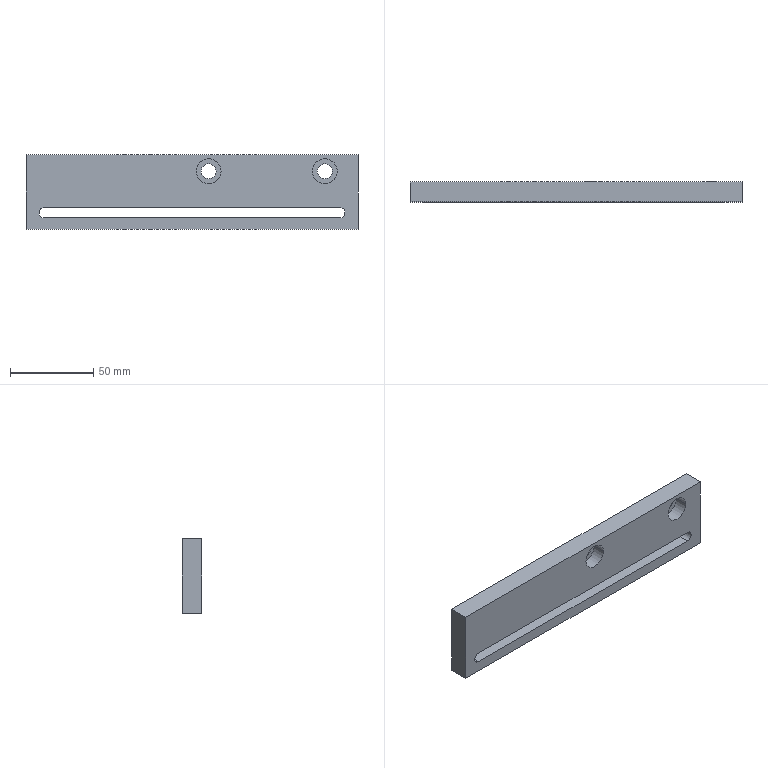Component | SolidWorks | SL021-102-4096.SL4PRT-1 | 1 solid | 21 faces | box 200 x 12 x 45 mm | volume 90833 mm3 | cylinder 11 | plane 10 | commonest cylinder face diameters 15 x4 9 x4 6.3 x3 | material AL6061
build123d program:
from build123d import *

# Parameters (mm, degrees)
SKETCH1_W                                          = 200
SKETCH1_H                                          = 45
BOSS_EXTRUDE1_DEPTH                                = 6
HOLE_SIZE_ACCORDING_TO_TYPE_1_OF_HEXAG_D           = 9
HOLE_SIZE_ACCORDING_TO_TYPE_1_OF_HEXAG_CBORE_D     = 15
HOLE_SIZE_ACCORDING_TO_TYPE_1_OF_HEXAG_CBORE_DEPTH = 8
CUT_EXTRUDE1_DEPTH                                 = 104.2


with BuildPart() as part:
    # Sketch1 → Boss-Extrude1 (new, symmetric)
    with BuildSketch(Plane.XY):
        Rectangle(SKETCH1_W, SKETCH1_H)
    extrude(amount=BOSS_EXTRUDE1_DEPTH, both=True)

    # Hole Size _According to_ Type 1 of Hexag (through all)
    with Locations(Plane(origin=(0, 0, 6), x_dir=(-1, 0, 0), z_dir=(0, 0, 1))):
        with Locations((-10, -12.5), (-80, -12.5)):
            CounterBoreHole(HOLE_SIZE_ACCORDING_TO_TYPE_1_OF_HEXAG_D / 2, HOLE_SIZE_ACCORDING_TO_TYPE_1_OF_HEXAG_CBORE_D / 2, HOLE_SIZE_ACCORDING_TO_TYPE_1_OF_HEXAG_CBORE_DEPTH)

    # Sketch4 → Cut-Extrude1 (cut, through all)
    with BuildSketch(Plane(origin=(0, 0, -6), x_dir=(-1, 0, 0), z_dir=(0, 0, -1))):
        with BuildLine():
            Line((-89, -9.35), (89, -9.35))
            ThreePointArc((89, -9.35), (92.15, -12.5), (89, -15.65))
            Line((89, -15.65), (-89, -15.65))
            ThreePointArc((-89, -15.65), (-92.15, -12.5), (-89, -9.35))
        make_face()
    extrude(amount=-CUT_EXTRUDE1_DEPTH, mode=Mode.SUBTRACT)


solid = part.part

# Placed as in the assembly
solid = solid.moved(Location((-136.163, -96.499, -318.878), (90, 0, 0)))
STEP:
#1=COLOUR_RGB('',0.7922,0.8196,0.9333);
#2=FILL_AREA_STYLE_COLOUR('',#1);
#3=FILL_AREA_STYLE('',(#2));
#4=SURFACE_STYLE_FILL_AREA(#3);
#5=SURFACE_SIDE_STYLE('',(#4));
#6=SURFACE_STYLE_USAGE(.BOTH.,#5);
#7=PRESENTATION_STYLE_ASSIGNMENT((#6));
#8=CARTESIAN_POINT('',(-8.989,-4.035,-13.046));
#9=VERTEX_POINT('',#8);
#10=CARTESIAN_POINT('',(-8.865,-4.035,-12.922));
#11=VERTEX_POINT('',#10);
#12=CARTESIAN_POINT('',(-8.865,-4.035,-13.046));
#13=DIRECTION('',(-0.,1.,-0.));
#14=DIRECTION('',(-1.,0.,0.));
#15=AXIS2_PLACEMENT_3D('',#12,#13,#14);
#16=CIRCLE('',#15,0.124);
#17=EDGE_CURVE('',#9,#11,#16,.T.);
#18=ORIENTED_EDGE('',*,*,#17,.F.);
#19=CARTESIAN_POINT('',(-8.989,-3.563,-13.046));
#20=VERTEX_POINT('',#19);
#21=CARTESIAN_POINT('',(-8.989,-4.035,-13.046));
#22=DIRECTION('',(-0.,1.,-0.));
#23=VECTOR('',#22,39.37);
#24=LINE('',#21,#23);
#25=EDGE_CURVE('',#9,#20,#24,.T.);
#26=ORIENTED_EDGE('',*,*,#25,.T.);
#27=CARTESIAN_POINT('',(-8.865,-3.563,-12.922));
#28=VERTEX_POINT('',#27);
#29=CARTESIAN_POINT('',(-8.865,-3.563,-13.046));
#30=DIRECTION('',(-0.,1.,-0.));
#31=DIRECTION('',(-1.,0.,0.));
#32=AXIS2_PLACEMENT_3D('',#29,#30,#31);
#33=CIRCLE('',#32,0.124);
#34=EDGE_CURVE('',#20,#28,#33,.T.);
#35=ORIENTED_EDGE('',*,*,#34,.T.);
#36=CARTESIAN_POINT('',(-8.865,-4.035,-12.922));
#37=DIRECTION('',(-0.,1.,-0.));
#38=VECTOR('',#37,39.37);
#39=LINE('',#36,#38);
#40=EDGE_CURVE('',#11,#28,#39,.T.);
#41=ORIENTED_EDGE('',*,*,#40,.F.);
#42=EDGE_LOOP('',(#18,#26,#35,#41));
#43=FACE_OUTER_BOUND('',#42,.T.);
#44=CARTESIAN_POINT('',(-8.865,-4.035,-13.046));
#45=DIRECTION('',(-0.,1.,-0.));
#46=DIRECTION('',(-1.,0.,0.));
#47=AXIS2_PLACEMENT_3D('',#44,#45,#46);
#48=CYLINDRICAL_SURFACE('',#47,0.124);
#49=ADVANCED_FACE('',(#43),#48,.F.);
#50=CARTESIAN_POINT('',(-5.262,-3.72,-12.062));
#51=VERTEX_POINT('',#50);
#52=CARTESIAN_POINT('',(-4.672,-3.72,-12.062));
#53=VERTEX_POINT('',#52);
#54=CARTESIAN_POINT('',(-4.967,-3.72,-12.062));
#55=DIRECTION('',(0.,-1.,0.));
#56=DIRECTION('',(1.,0.,0.));
#57=AXIS2_PLACEMENT_3D('',#54,#55,#56);
#58=CIRCLE('',#57,0.2953);
#59=EDGE_CURVE('',#51,#53,#58,.T.);
#60=ORIENTED_EDGE('',*,*,#59,.F.);
#61=CARTESIAN_POINT('',(-5.262,-4.035,-12.062));
#62=VERTEX_POINT('',#61);
#63=CARTESIAN_POINT('',(-5.262,-4.035,-12.062));
#64=DIRECTION('',(0.,-1.,0.));
#65=VECTOR('',#64,39.37);
#66=LINE('',#63,#65);
#67=EDGE_CURVE('',#51,#62,#66,.T.);
#68=ORIENTED_EDGE('',*,*,#67,.T.);
#69=CARTESIAN_POINT('',(-4.672,-4.035,-12.062));
#70=VERTEX_POINT('',#69);
#71=CARTESIAN_POINT('',(-4.967,-4.035,-12.062));
#72=DIRECTION('',(0.,-1.,0.));
#73=DIRECTION('',(1.,0.,0.));
#74=AXIS2_PLACEMENT_3D('',#71,#72,#73);
#75=CIRCLE('',#74,0.2953);
#76=EDGE_CURVE('',#62,#70,#75,.T.);
#77=ORIENTED_EDGE('',*,*,#76,.T.);
#78=CARTESIAN_POINT('',(-4.672,-4.035,-12.062));
#79=DIRECTION('',(0.,-1.,0.));
#80=VECTOR('',#79,39.37);
#81=LINE('',#78,#80);
#82=EDGE_CURVE('',#53,#70,#81,.T.);
#83=ORIENTED_EDGE('',*,*,#82,.F.);
#84=EDGE_LOOP('',(#60,#68,#77,#83));
#85=FACE_OUTER_BOUND('',#84,.T.);
#86=CARTESIAN_POINT('',(-4.967,-4.035,-12.062));
#87=DIRECTION('',(0.,-1.,0.));
#88=DIRECTION('',(1.,0.,0.));
#89=AXIS2_PLACEMENT_3D('',#86,#87,#88);
#90=CYLINDRICAL_SURFACE('',#89,0.2953);
#91=ADVANCED_FACE('',(#85),#90,.F.);
#92=CARTESIAN_POINT('',(-5.144,-3.563,-12.062));
#93=VERTEX_POINT('',#92);
#94=CARTESIAN_POINT('',(-4.79,-3.563,-12.062));
#95=VERTEX_POINT('',#94);
#96=CARTESIAN_POINT('',(-4.967,-3.563,-12.062));
#97=DIRECTION('',(0.,-1.,0.));
#98=DIRECTION('',(1.,0.,0.));
#99=AXIS2_PLACEMENT_3D('',#96,#97,#98);
#100=CIRCLE('',#99,0.1772);
#101=EDGE_CURVE('',#93,#95,#100,.T.);
#102=ORIENTED_EDGE('',*,*,#101,.F.);
#103=CARTESIAN_POINT('',(-5.144,-3.72,-12.062));
#104=VERTEX_POINT('',#103);
#105=CARTESIAN_POINT('',(-5.144,-4.035,-12.062));
#106=DIRECTION('',(0.,-1.,0.));
#107=VECTOR('',#106,39.37);
#108=LINE('',#105,#107);
#109=EDGE_CURVE('',#93,#104,#108,.T.);
#110=ORIENTED_EDGE('',*,*,#109,.T.);
#111=CARTESIAN_POINT('',(-4.79,-3.72,-12.062));
#112=VERTEX_POINT('',#111);
#113=CARTESIAN_POINT('',(-4.967,-3.72,-12.062));
#114=DIRECTION('',(0.,-1.,0.));
#115=DIRECTION('',(1.,0.,0.));
#116=AXIS2_PLACEMENT_3D('',#113,#114,#115);
#117=CIRCLE('',#116,0.1772);
#118=EDGE_CURVE('',#104,#112,#117,.T.);
#119=ORIENTED_EDGE('',*,*,#118,.T.);
#120=CARTESIAN_POINT('',(-4.79,-4.035,-12.062));
#121=DIRECTION('',(0.,-1.,0.));
#122=VECTOR('',#121,39.37);
#123=LINE('',#120,#122);
#124=EDGE_CURVE('',#95,#112,#123,.T.);
#125=ORIENTED_EDGE('',*,*,#124,.F.);
#126=EDGE_LOOP('',(#102,#110,#119,#125));
#127=FACE_OUTER_BOUND('',#126,.T.);
#128=CARTESIAN_POINT('',(-4.967,-4.035,-12.062));
#129=DIRECTION('',(0.,-1.,0.));
#130=DIRECTION('',(1.,0.,0.));
#131=AXIS2_PLACEMENT_3D('',#128,#129,#130);
#132=CYLINDRICAL_SURFACE('',#131,0.1772);
#133=ADVANCED_FACE('',(#127),#132,.F.);
#134=CARTESIAN_POINT('',(-2.506,-3.72,-12.062));
#135=VERTEX_POINT('',#134);
#136=CARTESIAN_POINT('',(-1.916,-3.72,-12.062));
#137=VERTEX_POINT('',#136);
#138=CARTESIAN_POINT('',(-2.211,-3.72,-12.062));
#139=DIRECTION('',(0.,-1.,0.));
#140=DIRECTION('',(1.,0.,0.));
#141=AXIS2_PLACEMENT_3D('',#138,#139,#140);
#142=CIRCLE('',#141,0.2953);
#143=EDGE_CURVE('',#135,#137,#142,.T.);
#144=ORIENTED_EDGE('',*,*,#143,.F.);
#145=CARTESIAN_POINT('',(-2.506,-4.035,-12.062));
#146=VERTEX_POINT('',#145);
#147=CARTESIAN_POINT('',(-2.506,-4.035,-12.062));
#148=DIRECTION('',(0.,-1.,0.));
#149=VECTOR('',#148,39.37);
#150=LINE('',#147,#149);
#151=EDGE_CURVE('',#135,#146,#150,.T.);
#152=ORIENTED_EDGE('',*,*,#151,.T.);
#153=CARTESIAN_POINT('',(-1.916,-4.035,-12.062));
#154=VERTEX_POINT('',#153);
#155=CARTESIAN_POINT('',(-2.211,-4.035,-12.062));
#156=DIRECTION('',(0.,-1.,0.));
#157=DIRECTION('',(1.,0.,0.));
#158=AXIS2_PLACEMENT_3D('',#155,#156,#157);
#159=CIRCLE('',#158,0.2953);
#160=EDGE_CURVE('',#146,#154,#159,.T.);
#161=ORIENTED_EDGE('',*,*,#160,.T.);
#162=CARTESIAN_POINT('',(-1.916,-4.035,-12.062));
#163=DIRECTION('',(0.,-1.,0.));
#164=VECTOR('',#163,39.37);
#165=LINE('',#162,#164);
#166=EDGE_CURVE('',#137,#154,#165,.T.);
#167=ORIENTED_EDGE('',*,*,#166,.F.);
#168=EDGE_LOOP('',(#144,#152,#161,#167));
#169=FACE_OUTER_BOUND('',#168,.T.);
#170=CARTESIAN_POINT('',(-2.211,-4.035,-12.062));
#171=DIRECTION('',(0.,-1.,0.));
#172=DIRECTION('',(1.,0.,0.));
#173=AXIS2_PLACEMENT_3D('',#170,#171,#172);
#174=CYLINDRICAL_SURFACE('',#173,0.2953);
#175=ADVANCED_FACE('',(#169),#174,.F.);
#176=CARTESIAN_POINT('',(-2.388,-3.563,-12.062));
#177=VERTEX_POINT('',#176);
#178=CARTESIAN_POINT('',(-2.034,-3.563,-12.062));
#179=VERTEX_POINT('',#178);
#180=CARTESIAN_POINT('',(-2.211,-3.563,-12.062));
#181=DIRECTION('',(0.,-1.,0.));
#182=DIRECTION('',(1.,0.,0.));
#183=AXIS2_PLACEMENT_3D('',#180,#181,#182);
#184=CIRCLE('',#183,0.1772);
#185=EDGE_CURVE('',#177,#179,#184,.T.);
#186=ORIENTED_EDGE('',*,*,#185,.F.);
#187=CARTESIAN_POINT('',(-2.388,-3.72,-12.062));
#188=VERTEX_POINT('',#187);
#189=CARTESIAN_POINT('',(-2.388,-4.035,-12.062));
#190=DIRECTION('',(0.,-1.,0.));
#191=VECTOR('',#190,39.37);
#192=LINE('',#189,#191);
#193=EDGE_CURVE('',#177,#188,#192,.T.);
#194=ORIENTED_EDGE('',*,*,#193,.T.);
#195=CARTESIAN_POINT('',(-2.034,-3.72,-12.062));
#196=VERTEX_POINT('',#195);
#197=CARTESIAN_POINT('',(-2.211,-3.72,-12.062));
#198=DIRECTION('',(0.,-1.,0.));
#199=DIRECTION('',(1.,0.,0.));
#200=AXIS2_PLACEMENT_3D('',#197,#198,#199);
#201=CIRCLE('',#200,0.1772);
#202=EDGE_CURVE('',#188,#196,#201,.T.);
#203=ORIENTED_EDGE('',*,*,#202,.T.);
#204=CARTESIAN_POINT('',(-2.034,-4.035,-12.062));
#205=DIRECTION('',(0.,-1.,0.));
#206=VECTOR('',#205,39.37);
#207=LINE('',#204,#206);
#208=EDGE_CURVE('',#179,#196,#207,.T.);
#209=ORIENTED_EDGE('',*,*,#208,.F.);
#210=EDGE_LOOP('',(#186,#194,#203,#209));
#211=FACE_OUTER_BOUND('',#210,.T.);
#212=CARTESIAN_POINT('',(-2.211,-4.035,-12.062));
#213=DIRECTION('',(0.,-1.,0.));
#214=DIRECTION('',(1.,0.,0.));
#215=AXIS2_PLACEMENT_3D('',#212,#213,#214);
#216=CYLINDRICAL_SURFACE('',#215,0.1772);
#217=ADVANCED_FACE('',(#211),#216,.F.);
#218=CARTESIAN_POINT('',(-1.424,-3.563,-13.44));
#219=VERTEX_POINT('',#218);
#220=CARTESIAN_POINT('',(-1.424,-3.563,-11.668));
#221=VERTEX_POINT('',#220);
#222=CARTESIAN_POINT('',(-1.424,-3.563,-13.44));
#223=DIRECTION('',(-0.,0.,1.));
#224=VECTOR('',#223,39.37);
#225=LINE('',#222,#224);
#226=EDGE_CURVE('',#219,#221,#225,.T.);
#227=ORIENTED_EDGE('',*,*,#226,.T.);
#228=CARTESIAN_POINT('',(-1.424,-4.035,-11.668));
#229=VERTEX_POINT('',#228);
#230=CARTESIAN_POINT('',(-1.424,-4.035,-11.668));
#231=DIRECTION('',(-0.,1.,-0.));
#232=VECTOR('',#231,39.37);
#233=LINE('',#230,#232);
#234=EDGE_CURVE('',#229,#221,#233,.T.);
#235=ORIENTED_EDGE('',*,*,#234,.F.);
#236=CARTESIAN_POINT('',(-1.424,-4.035,-13.44));
#237=VERTEX_POINT('',#236);
#238=CARTESIAN_POINT('',(-1.424,-4.035,-13.44));
#239=DIRECTION('',(-0.,0.,1.));
#240=VECTOR('',#239,39.37);
#241=LINE('',#238,#240);
#242=EDGE_CURVE('',#237,#229,#241,.T.);
#243=ORIENTED_EDGE('',*,*,#242,.F.);
#244=CARTESIAN_POINT('',(-1.424,-4.035,-13.44));
#245=DIRECTION('',(-0.,1.,-0.));
#246=VECTOR('',#245,39.37);
#247=LINE('',#244,#246);
#248=EDGE_CURVE('',#237,#219,#247,.T.);
#249=ORIENTED_EDGE('',*,*,#248,.T.);
#250=EDGE_LOOP('',(#227,#235,#243,#249));
#251=FACE_OUTER_BOUND('',#250,.T.);
#252=CARTESIAN_POINT('',(-1.424,-4.035,-13.44));
#253=DIRECTION('',(-1.,-0.,-0.));
#254=DIRECTION('',(0.,-1.,0.));
#255=AXIS2_PLACEMENT_3D('',#252,#253,#254);
#256=PLANE('',#255);
#257=ADVANCED_FACE('',(#251),#256,.F.);
#258=CARTESIAN_POINT('',(-9.298,-3.563,-11.668));
#259=VERTEX_POINT('',#258);
#260=CARTESIAN_POINT('',(-9.298,-3.563,-11.668));
#261=DIRECTION('',(-1.,-0.,-0.));
#262=VECTOR('',#261,39.37);
#263=LINE('',#260,#262);
#264=EDGE_CURVE('',#221,#259,#263,.T.);
#265=ORIENTED_EDGE('',*,*,#264,.T.);
#266=CARTESIAN_POINT('',(-9.298,-4.035,-11.668));
#267=VERTEX_POINT('',#266);
#268=CARTESIAN_POINT('',(-9.298,-4.035,-11.668));
#269=DIRECTION('',(-0.,1.,-0.));
#270=VECTOR('',#269,39.37);
#271=LINE('',#268,#270);
#272=EDGE_CURVE('',#267,#259,#271,.T.);
#273=ORIENTED_EDGE('',*,*,#272,.F.);
#274=CARTESIAN_POINT('',(-9.298,-4.035,-11.668));
#275=DIRECTION('',(-1.,-0.,-0.));
#276=VECTOR('',#275,39.37);
#277=LINE('',#274,#276);
#278=EDGE_CURVE('',#229,#267,#277,.T.);
#279=ORIENTED_EDGE('',*,*,#278,.F.);
#280=ORIENTED_EDGE('',*,*,#234,.T.);
#281=EDGE_LOOP('',(#265,#273,#279,#280));
#282=FACE_OUTER_BOUND('',#281,.T.);
#283=CARTESIAN_POINT('',(-9.298,-4.035,-11.668));
#284=DIRECTION('',(0.,-0.,-1.));
#285=DIRECTION('',(-0.,1.,-0.));
#286=AXIS2_PLACEMENT_3D('',#283,#284,#285);
#287=PLANE('',#286);
#288=ADVANCED_FACE('',(#282),#287,.F.);
#289=CARTESIAN_POINT('',(-9.298,-3.563,-13.44));
#290=VERTEX_POINT('',#289);
#291=CARTESIAN_POINT('',(-9.298,-3.563,-13.44));
#292=DIRECTION('',(0.,-0.,-1.));
#293=VECTOR('',#292,39.37);
#294=LINE('',#291,#293);
#295=EDGE_CURVE('',#259,#290,#294,.T.);
#296=ORIENTED_EDGE('',*,*,#295,.T.);
#297=CARTESIAN_POINT('',(-9.298,-4.035,-13.44));
#298=VERTEX_POINT('',#297);
#299=CARTESIAN_POINT('',(-9.298,-4.035,-13.44));
#300=DIRECTION('',(-0.,1.,-0.));
#301=VECTOR('',#300,39.37);
#302=LINE('',#299,#301);
#303=EDGE_CURVE('',#298,#290,#302,.T.);
#304=ORIENTED_EDGE('',*,*,#303,.F.);
#305=CARTESIAN_POINT('',(-9.298,-4.035,-13.44));
#306=DIRECTION('',(0.,-0.,-1.));
#307=VECTOR('',#306,39.37);
#308=LINE('',#305,#307);
#309=EDGE_CURVE('',#267,#298,#308,.T.);
#310=ORIENTED_EDGE('',*,*,#309,.F.);
#311=ORIENTED_EDGE('',*,*,#272,.T.);
#312=EDGE_LOOP('',(#296,#304,#310,#311));
#313=FACE_OUTER_BOUND('',#312,.T.);
#314=CARTESIAN_POINT('',(-9.298,-4.035,-13.44));
#315=DIRECTION('',(1.,0.,0.));
#316=DIRECTION('',(-0.,1.,-0.));
#317=AXIS2_PLACEMENT_3D('',#314,#315,#316);
#318=PLANE('',#317);
#319=ADVANCED_FACE('',(#313),#318,.F.);
#320=CARTESIAN_POINT('',(-9.298,-3.563,-13.44));
#321=DIRECTION('',(1.,0.,0.));
#322=VECTOR('',#321,39.37);
#323=LINE('',#320,#322);
#324=EDGE_CURVE('',#290,#219,#323,.T.);
#325=ORIENTED_EDGE('',*,*,#324,.T.);
#326=ORIENTED_EDGE('',*,*,#248,.F.);
#327=CARTESIAN_POINT('',(-9.298,-4.035,-13.44));
#328=DIRECTION('',(1.,0.,0.));
#329=VECTOR('',#328,39.37);
#330=LINE('',#327,#329);
#331=EDGE_CURVE('',#298,#237,#330,.T.);
#332=ORIENTED_EDGE('',*,*,#331,.F.);
#333=ORIENTED_EDGE('',*,*,#303,.T.);
#334=EDGE_LOOP('',(#325,#326,#332,#333));
#335=FACE_OUTER_BOUND('',#334,.T.);
#336=CARTESIAN_POINT('',(-9.298,-4.035,-13.44));
#337=DIRECTION('',(-0.,0.,1.));
#338=DIRECTION('',(0.,-1.,0.));
#339=AXIS2_PLACEMENT_3D('',#336,#337,#338);
#340=PLANE('',#339);
#341=ADVANCED_FACE('',(#335),#340,.F.);
#342=CARTESIAN_POINT('',(-1.857,-4.035,-12.922));
#343=VERTEX_POINT('',#342);
#344=CARTESIAN_POINT('',(-1.857,-4.035,-12.922));
#345=DIRECTION('',(1.,0.,0.));
#346=VECTOR('',#345,39.37);
#347=LINE('',#344,#346);
#348=EDGE_CURVE('',#11,#343,#347,.T.);
#349=ORIENTED_EDGE('',*,*,#348,.T.);
#350=CARTESIAN_POINT('',(-1.857,-4.035,-13.17));
#351=VERTEX_POINT('',#350);
#352=CARTESIAN_POINT('',(-1.857,-4.035,-13.046));
#353=DIRECTION('',(-0.,1.,-0.));
#354=DIRECTION('',(-1.,0.,0.));
#355=AXIS2_PLACEMENT_3D('',#352,#353,#354);
#356=CIRCLE('',#355,0.124);
#357=EDGE_CURVE('',#343,#351,#356,.T.);
#358=ORIENTED_EDGE('',*,*,#357,.T.);
#359=CARTESIAN_POINT('',(-8.865,-4.035,-13.17));
#360=VERTEX_POINT('',#359);
#361=CARTESIAN_POINT('',(-1.857,-4.035,-13.17));
#362=DIRECTION('',(-1.,-0.,-0.));
#363=VECTOR('',#362,39.37);
#364=LINE('',#361,#363);
#365=EDGE_CURVE('',#351,#360,#364,.T.);
#366=ORIENTED_EDGE('',*,*,#365,.T.);
#367=CARTESIAN_POINT('',(-8.865,-4.035,-13.046));
#368=DIRECTION('',(-0.,1.,-0.));
#369=DIRECTION('',(-1.,0.,0.));
#370=AXIS2_PLACEMENT_3D('',#367,#368,#369);
#371=CIRCLE('',#370,0.124);
#372=EDGE_CURVE('',#360,#9,#371,.T.);
#373=ORIENTED_EDGE('',*,*,#372,.T.);
#374=ORIENTED_EDGE('',*,*,#17,.T.);
#375=EDGE_LOOP('',(#349,#358,#366,#373,#374));
#376=FACE_BOUND('',#375,.T.);
#377=CARTESIAN_POINT('',(-4.967,-4.035,-12.062));
#378=DIRECTION('',(0.,-1.,0.));
#379=DIRECTION('',(1.,0.,0.));
#380=AXIS2_PLACEMENT_3D('',#377,#378,#379);
#381=CIRCLE('',#380,0.2953);
#382=EDGE_CURVE('',#70,#62,#381,.T.);
#383=ORIENTED_EDGE('',*,*,#382,.F.);
#384=ORIENTED_EDGE('',*,*,#76,.F.);
#385=EDGE_LOOP('',(#383,#384));
#386=FACE_BOUND('',#385,.T.);
#387=CARTESIAN_POINT('',(-2.211,-4.035,-12.062));
#388=DIRECTION('',(0.,-1.,0.));
#389=DIRECTION('',(1.,0.,0.));
#390=AXIS2_PLACEMENT_3D('',#387,#388,#389);
#391=CIRCLE('',#390,0.2953);
#392=EDGE_CURVE('',#154,#146,#391,.T.);
#393=ORIENTED_EDGE('',*,*,#392,.F.);
#394=ORIENTED_EDGE('',*,*,#160,.F.);
#395=EDGE_LOOP('',(#393,#394));
#396=FACE_BOUND('',#395,.T.);
#397=ORIENTED_EDGE('',*,*,#242,.T.);
#398=ORIENTED_EDGE('',*,*,#278,.T.);
#399=ORIENTED_EDGE('',*,*,#309,.T.);
#400=ORIENTED_EDGE('',*,*,#331,.T.);
#401=EDGE_LOOP('',(#397,#398,#399,#400));
#402=FACE_OUTER_BOUND('',#401,.T.);
#403=CARTESIAN_POINT('',(-5.361,-4.035,-12.554));
#404=DIRECTION('',(-0.,1.,-0.));
#405=DIRECTION('',(-1.,-0.,-0.));
#406=AXIS2_PLACEMENT_3D('',#403,#404,#405);
#407=PLANE('',#406);
#408=ADVANCED_FACE('',(#376,#386,#396,#402),#407,.F.);
#409=CARTESIAN_POINT('',(-1.857,-3.563,-12.922));
#410=VERTEX_POINT('',#409);
#411=CARTESIAN_POINT('',(-1.857,-3.563,-13.17));
#412=VERTEX_POINT('',#411);
#413=CARTESIAN_POINT('',(-1.857,-3.563,-13.046));
#414=DIRECTION('',(-0.,1.,-0.));
#415=DIRECTION('',(-1.,0.,0.));
#416=AXIS2_PLACEMENT_3D('',#413,#414,#415);
#417=CIRCLE('',#416,0.124);
#418=EDGE_CURVE('',#410,#412,#417,.T.);
#419=ORIENTED_EDGE('',*,*,#418,.F.);
#420=CARTESIAN_POINT('',(-1.857,-3.563,-12.922));
#421=DIRECTION('',(1.,0.,0.));
#422=VECTOR('',#421,39.37);
#423=LINE('',#420,#422);
#424=EDGE_CURVE('',#28,#410,#423,.T.);
#425=ORIENTED_EDGE('',*,*,#424,.F.);
#426=ORIENTED_EDGE('',*,*,#34,.F.);
#427=CARTESIAN_POINT('',(-8.865,-3.563,-13.17));
#428=VERTEX_POINT('',#427);
#429=CARTESIAN_POINT('',(-8.865,-3.563,-13.046));
#430=DIRECTION('',(-0.,1.,-0.));
#431=DIRECTION('',(-1.,0.,0.));
#432=AXIS2_PLACEMENT_3D('',#429,#430,#431);
#433=CIRCLE('',#432,0.124);
#434=EDGE_CURVE('',#428,#20,#433,.T.);
#435=ORIENTED_EDGE('',*,*,#434,.F.);
#436=CARTESIAN_POINT('',(-1.857,-3.563,-13.17));
#437=DIRECTION('',(-1.,-0.,-0.));
#438=VECTOR('',#437,39.37);
#439=LINE('',#436,#438);
#440=EDGE_CURVE('',#412,#428,#439,.T.);
#441=ORIENTED_EDGE('',*,*,#440,.F.);
#442=EDGE_LOOP('',(#419,#425,#426,#435,#441));
#443=FACE_BOUND('',#442,.T.);
#444=CARTESIAN_POINT('',(-4.967,-3.563,-12.062));
#445=DIRECTION('',(0.,-1.,0.));
#446=DIRECTION('',(1.,0.,0.));
#447=AXIS2_PLACEMENT_3D('',#444,#445,#446);
#448=CIRCLE('',#447,0.1772);
#449=EDGE_CURVE('',#95,#93,#448,.T.);
#450=ORIENTED_EDGE('',*,*,#449,.T.);
#451=ORIENTED_EDGE('',*,*,#101,.T.);
#452=EDGE_LOOP('',(#450,#451));
#453=FACE_BOUND('',#452,.T.);
#454=CARTESIAN_POINT('',(-2.211,-3.563,-12.062));
#455=DIRECTION('',(0.,-1.,0.));
#456=DIRECTION('',(1.,0.,0.));
#457=AXIS2_PLACEMENT_3D('',#454,#455,#456);
#458=CIRCLE('',#457,0.1772);
#459=EDGE_CURVE('',#179,#177,#458,.T.);
#460=ORIENTED_EDGE('',*,*,#459,.T.);
#461=ORIENTED_EDGE('',*,*,#185,.T.);
#462=EDGE_LOOP('',(#460,#461));
#463=FACE_BOUND('',#462,.T.);
#464=ORIENTED_EDGE('',*,*,#226,.F.);
#465=ORIENTED_EDGE('',*,*,#324,.F.);
#466=ORIENTED_EDGE('',*,*,#295,.F.);
#467=ORIENTED_EDGE('',*,*,#264,.F.);
#468=EDGE_LOOP('',(#464,#465,#466,#467));
#469=FACE_OUTER_BOUND('',#468,.T.);
#470=CARTESIAN_POINT('',(-5.361,-3.563,-12.554));
#471=DIRECTION('',(-0.,1.,-0.));
#472=DIRECTION('',(-1.,-0.,-0.));
#473=AXIS2_PLACEMENT_3D('',#470,#471,#472);
#474=PLANE('',#473);
#475=ADVANCED_FACE('',(#443,#453,#463,#469),#474,.T.);
#476=ORIENTED_EDGE('',*,*,#193,.F.);
#477=ORIENTED_EDGE('',*,*,#459,.F.);
#478=ORIENTED_EDGE('',*,*,#208,.T.);
#479=CARTESIAN_POINT('',(-2.211,-3.72,-12.062));
#480=DIRECTION('',(0.,-1.,0.));
#481=DIRECTION('',(1.,0.,0.));
#482=AXIS2_PLACEMENT_3D('',#479,#480,#481);
#483=CIRCLE('',#482,0.1772);
#484=EDGE_CURVE('',#196,#188,#483,.T.);
#485=ORIENTED_EDGE('',*,*,#484,.T.);
#486=EDGE_LOOP('',(#476,#477,#478,#485));
#487=FACE_OUTER_BOUND('',#486,.T.);
#488=CARTESIAN_POINT('',(-2.211,-4.035,-12.062));
#489=DIRECTION('',(0.,-1.,0.));
#490=DIRECTION('',(1.,0.,0.));
#491=AXIS2_PLACEMENT_3D('',#488,#489,#490);
#492=CYLINDRICAL_SURFACE('',#491,0.1772);
#493=ADVANCED_FACE('',(#487),#492,.F.);
#494=ORIENTED_EDGE('',*,*,#484,.F.);
#495=ORIENTED_EDGE('',*,*,#202,.F.);
#496=EDGE_LOOP('',(#494,#495));
#497=FACE_BOUND('',#496,.T.);
#498=CARTESIAN_POINT('',(-2.211,-3.72,-12.062));
#499=DIRECTION('',(0.,-1.,0.));
#500=DIRECTION('',(1.,0.,0.));
#501=AXIS2_PLACEMENT_3D('',#498,#499,#500);
#502=CIRCLE('',#501,0.2953);
#503=EDGE_CURVE('',#137,#135,#502,.T.);
#504=ORIENTED_EDGE('',*,*,#503,.T.);
#505=ORIENTED_EDGE('',*,*,#143,.T.);
#506=EDGE_LOOP('',(#504,#505));
#507=FACE_OUTER_BOUND('',#506,.T.);
#508=CARTESIAN_POINT('',(-2.034,-3.72,-12.062));
#509=DIRECTION('',(-0.,1.,-0.));
#510=DIRECTION('',(-1.,-0.,-0.));
#511=AXIS2_PLACEMENT_3D('',#508,#509,#510);
#512=PLANE('',#511);
#513=ADVANCED_FACE('',(#497,#507),#512,.F.);
#514=ORIENTED_EDGE('',*,*,#151,.F.);
#515=ORIENTED_EDGE('',*,*,#503,.F.);
#516=ORIENTED_EDGE('',*,*,#166,.T.);
#517=ORIENTED_EDGE('',*,*,#392,.T.);
#518=EDGE_LOOP('',(#514,#515,#516,#517));
#519=FACE_OUTER_BOUND('',#518,.T.);
#520=CARTESIAN_POINT('',(-2.211,-4.035,-12.062));
#521=DIRECTION('',(0.,-1.,0.));
#522=DIRECTION('',(1.,0.,0.));
#523=AXIS2_PLACEMENT_3D('',#520,#521,#522);
#524=CYLINDRICAL_SURFACE('',#523,0.2953);
#525=ADVANCED_FACE('',(#519),#524,.F.);
#526=ORIENTED_EDGE('',*,*,#109,.F.);
#527=ORIENTED_EDGE('',*,*,#449,.F.);
#528=ORIENTED_EDGE('',*,*,#124,.T.);
#529=CARTESIAN_POINT('',(-4.967,-3.72,-12.062));
#530=DIRECTION('',(0.,-1.,0.));
#531=DIRECTION('',(1.,0.,0.));
#532=AXIS2_PLACEMENT_3D('',#529,#530,#531);
#533=CIRCLE('',#532,0.1772);
#534=EDGE_CURVE('',#112,#104,#533,.T.);
#535=ORIENTED_EDGE('',*,*,#534,.T.);
#536=EDGE_LOOP('',(#526,#527,#528,#535));
#537=FACE_OUTER_BOUND('',#536,.T.);
#538=CARTESIAN_POINT('',(-4.967,-4.035,-12.062));
#539=DIRECTION('',(0.,-1.,0.));
#540=DIRECTION('',(1.,0.,0.));
#541=AXIS2_PLACEMENT_3D('',#538,#539,#540);
#542=CYLINDRICAL_SURFACE('',#541,0.1772);
#543=ADVANCED_FACE('',(#537),#542,.F.);
#544=ORIENTED_EDGE('',*,*,#534,.F.);
#545=ORIENTED_EDGE('',*,*,#118,.F.);
#546=EDGE_LOOP('',(#544,#545));
#547=FACE_BOUND('',#546,.T.);
#548=CARTESIAN_POINT('',(-4.967,-3.72,-12.062));
#549=DIRECTION('',(0.,-1.,0.));
#550=DIRECTION('',(1.,0.,0.));
#551=AXIS2_PLACEMENT_3D('',#548,#549,#550);
#552=CIRCLE('',#551,0.2953);
#553=EDGE_CURVE('',#53,#51,#552,.T.);
#554=ORIENTED_EDGE('',*,*,#553,.T.);
#555=ORIENTED_EDGE('',*,*,#59,.T.);
#556=EDGE_LOOP('',(#554,#555));
#557=FACE_OUTER_BOUND('',#556,.T.);
#558=CARTESIAN_POINT('',(-4.79,-3.72,-12.062));
#559=DIRECTION('',(-0.,1.,-0.));
#560=DIRECTION('',(-1.,-0.,-0.));
#561=AXIS2_PLACEMENT_3D('',#558,#559,#560);
#562=PLANE('',#561);
#563=ADVANCED_FACE('',(#547,#557),#562,.F.);
#564=ORIENTED_EDGE('',*,*,#67,.F.);
#565=ORIENTED_EDGE('',*,*,#553,.F.);
#566=ORIENTED_EDGE('',*,*,#82,.T.);
#567=ORIENTED_EDGE('',*,*,#382,.T.);
#568=EDGE_LOOP('',(#564,#565,#566,#567));
#569=FACE_OUTER_BOUND('',#568,.T.);
#570=CARTESIAN_POINT('',(-4.967,-4.035,-12.062));
#571=DIRECTION('',(0.,-1.,0.));
#572=DIRECTION('',(1.,0.,0.));
#573=AXIS2_PLACEMENT_3D('',#570,#571,#572);
#574=CYLINDRICAL_SURFACE('',#573,0.2953);
#575=ADVANCED_FACE('',(#569),#574,.F.);
#576=ORIENTED_EDGE('',*,*,#418,.T.);
#577=CARTESIAN_POINT('',(-1.857,-4.035,-13.17));
#578=DIRECTION('',(-0.,1.,-0.));
#579=VECTOR('',#578,39.37);
#580=LINE('',#577,#579);
#581=EDGE_CURVE('',#351,#412,#580,.T.);
#582=ORIENTED_EDGE('',*,*,#581,.F.);
#583=ORIENTED_EDGE('',*,*,#357,.F.);
#584=CARTESIAN_POINT('',(-1.857,-4.035,-12.922));
#585=DIRECTION('',(-0.,1.,-0.));
#586=VECTOR('',#585,39.37);
#587=LINE('',#584,#586);
#588=EDGE_CURVE('',#343,#410,#587,.T.);
#589=ORIENTED_EDGE('',*,*,#588,.T.);
#590=EDGE_LOOP('',(#576,#582,#583,#589));
#591=FACE_OUTER_BOUND('',#590,.T.);
#592=CARTESIAN_POINT('',(-1.857,-4.035,-13.046));
#593=DIRECTION('',(-0.,1.,-0.));
#594=DIRECTION('',(-1.,0.,0.));
#595=AXIS2_PLACEMENT_3D('',#592,#593,#594);
#596=CYLINDRICAL_SURFACE('',#595,0.124);
#597=ADVANCED_FACE('',(#591),#596,.F.);
#598=ORIENTED_EDGE('',*,*,#424,.T.);
#599=ORIENTED_EDGE('',*,*,#588,.F.);
#600=ORIENTED_EDGE('',*,*,#348,.F.);
#601=ORIENTED_EDGE('',*,*,#40,.T.);
#602=EDGE_LOOP('',(#598,#599,#600,#601));
#603=FACE_OUTER_BOUND('',#602,.T.);
#604=CARTESIAN_POINT('',(-1.857,-4.035,-12.922));
#605=DIRECTION('',(-0.,0.,1.));
#606=DIRECTION('',(0.,-1.,0.));
#607=AXIS2_PLACEMENT_3D('',#604,#605,#606);
#608=PLANE('',#607);
#609=ADVANCED_FACE('',(#603),#608,.F.);
#610=ORIENTED_EDGE('',*,*,#25,.F.);
#611=ORIENTED_EDGE('',*,*,#372,.F.);
#612=CARTESIAN_POINT('',(-8.865,-4.035,-13.17));
#613=DIRECTION('',(-0.,1.,-0.));
#614=VECTOR('',#613,39.37);
#615=LINE('',#612,#614);
#616=EDGE_CURVE('',#360,#428,#615,.T.);
#617=ORIENTED_EDGE('',*,*,#616,.T.);
#618=ORIENTED_EDGE('',*,*,#434,.T.);
#619=EDGE_LOOP('',(#610,#611,#617,#618));
#620=FACE_OUTER_BOUND('',#619,.T.);
#621=CARTESIAN_POINT('',(-8.865,-4.035,-13.046));
#622=DIRECTION('',(-0.,1.,-0.));
#623=DIRECTION('',(-1.,0.,0.));
#624=AXIS2_PLACEMENT_3D('',#621,#622,#623);
#625=CYLINDRICAL_SURFACE('',#624,0.124);
#626=ADVANCED_FACE('',(#620),#625,.F.);
#627=ORIENTED_EDGE('',*,*,#440,.T.);
#628=ORIENTED_EDGE('',*,*,#616,.F.);
#629=ORIENTED_EDGE('',*,*,#365,.F.);
#630=ORIENTED_EDGE('',*,*,#581,.T.);
#631=EDGE_LOOP('',(#627,#628,#629,#630));
#632=FACE_OUTER_BOUND('',#631,.T.);
#633=CARTESIAN_POINT('',(-1.857,-4.035,-13.17));
#634=DIRECTION('',(0.,-0.,-1.));
#635=DIRECTION('',(-0.,1.,-0.));
#636=AXIS2_PLACEMENT_3D('',#633,#634,#635);
#637=PLANE('',#636);
#638=ADVANCED_FACE('',(#632),#637,.F.);
#639=CLOSED_SHELL('',(#49,#91,#133,#175,#217,#257,#288,#319,#341,#408,#475,#493,#513,#525,#543,#563,#575,#597,#609,#626,#638));
#640=MANIFOLD_SOLID_BREP('',#639);
#641=STYLED_ITEM('',(#7),#640);
#642=PRESENTATION_LAYER_ASSIGNMENT('','',(#641));
#643=CARTESIAN_POINT('',(0.,0.,0.));
#644=DIRECTION('',(0.,0.,1.));
#645=DIRECTION('',(1.,0.,0.));
#646=AXIS2_PLACEMENT_3D('',#643,#644,#645);
#647=(LENGTH_UNIT()NAMED_UNIT(*)SI_UNIT($,.METRE.));
#648=LENGTH_MEASURE_WITH_UNIT(LENGTH_MEASURE(0.0254),#647);
#649=DIMENSIONAL_EXPONENTS(1.,0.,0.,0.,0.,0.,0.);
#650=(CONVERSION_BASED_UNIT('',#648)LENGTH_UNIT()NAMED_UNIT(#649));
#651=UNCERTAINTY_MEASURE_WITH_UNIT(LENGTH_MEASURE(0.00001),#650,'','');
#652=(NAMED_UNIT(*)PLANE_ANGLE_UNIT()SI_UNIT($,.RADIAN.));
#653=(NAMED_UNIT(*)SI_UNIT($,.STERADIAN.)SOLID_ANGLE_UNIT());
#654=(GEOMETRIC_REPRESENTATION_CONTEXT(3)GLOBAL_UNCERTAINTY_ASSIGNED_CONTEXT((#651))GLOBAL_UNIT_ASSIGNED_CONTEXT((#650,#652,#653))REPRESENTATION_CONTEXT('',''));
#655=ADVANCED_BREP_SHAPE_REPRESENTATION('',(#640,#646),#654);
#656=(LENGTH_UNIT()NAMED_UNIT(*)SI_UNIT($,.METRE.));
#657=LENGTH_MEASURE_WITH_UNIT(LENGTH_MEASURE(0.0254),#656);
#658=DIMENSIONAL_EXPONENTS(1.,0.,0.,0.,0.,0.,0.);
#659=(CONVERSION_BASED_UNIT('',#657)LENGTH_UNIT()NAMED_UNIT(#658));
#660=UNCERTAINTY_MEASURE_WITH_UNIT(LENGTH_MEASURE(0.00001),#659,'','');
#661=(NAMED_UNIT(*)PLANE_ANGLE_UNIT()SI_UNIT($,.RADIAN.));
#662=(NAMED_UNIT(*)SI_UNIT($,.STERADIAN.)SOLID_ANGLE_UNIT());
#663=(GEOMETRIC_REPRESENTATION_CONTEXT(3)GLOBAL_UNCERTAINTY_ASSIGNED_CONTEXT((#660))GLOBAL_UNIT_ASSIGNED_CONTEXT((#659,#661,#662))REPRESENTATION_CONTEXT('',''));
#664=MECHANICAL_DESIGN_GEOMETRIC_PRESENTATION_REPRESENTATION('',(#641),#663);